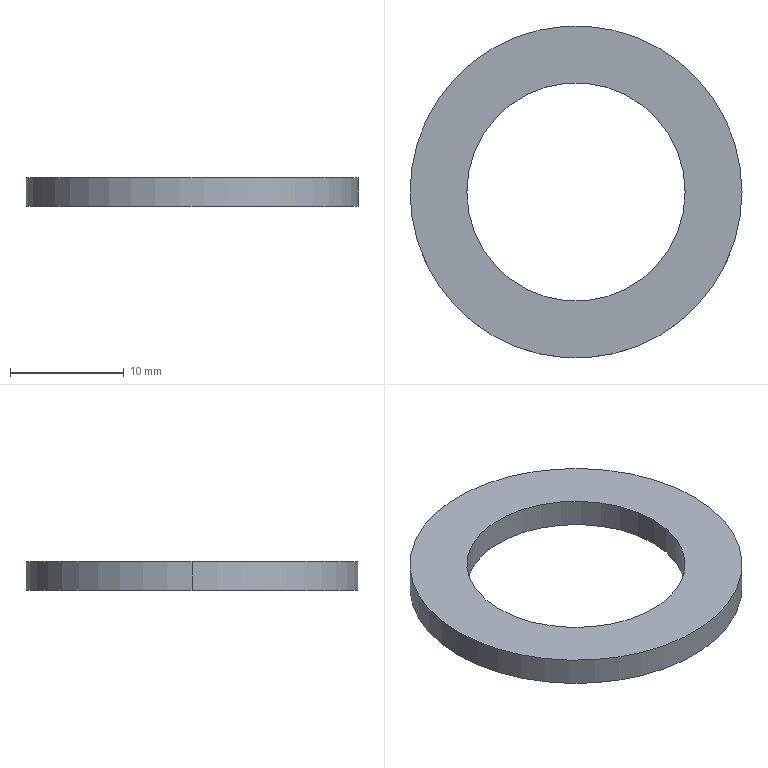Component | SolidWorks | TractionDrivenWheel-1_BearingPlate2-1 | 1 solid | 6 faces | box 29.2 x 29.2 x 2.5 mm | volume 950 mm3 | cylinder 4 | plane 2 | commonest cylinder face diameters 19.2 x2 29.2 x2
build123d program:
from build123d import *

# Parameters (mm, degrees)
SKETCH1_R           = 14.6
SKETCH1_R_2         = 9.6
BOSS_EXTRUDE1_DEPTH = 2.5


with BuildPart() as part:
    # Sketch1 → Boss-Extrude1 (new body)
    with BuildSketch(Plane(origin=(0, 0, 0), x_dir=(0, 0, -1), z_dir=(1, 0, 0))):
        Circle(SKETCH1_R)
        Circle(SKETCH1_R_2, mode=Mode.SUBTRACT)
    extrude(amount=BOSS_EXTRUDE1_DEPTH)


solid = part.part

# Placed as in the assembly
solid = solid.moved(Location((225.493, -197.911, 521), (0, 90, 0)))
STEP:
#1=CARTESIAN_POINT('',(9.256,-7.792,20.413));
#2=VERTEX_POINT('',#1);
#3=CARTESIAN_POINT('',(8.5,-7.792,20.413));
#4=VERTEX_POINT('',#3);
#5=CARTESIAN_POINT('',(8.878,-7.792,20.413));
#6=DIRECTION('',(0.,0.,-1.));
#7=DIRECTION('',(-1.,0.,0.));
#8=AXIS2_PLACEMENT_3D('',#5,#6,#7);
#9=CIRCLE('',#8,0.378);
#10=EDGE_CURVE('',#2,#4,#9,.T.);
#11=ORIENTED_EDGE('',*,*,#10,.T.);
#12=CARTESIAN_POINT('',(8.5,-7.792,20.512));
#13=VERTEX_POINT('',#12);
#14=CARTESIAN_POINT('',(8.5,-7.792,20.413));
#15=DIRECTION('',(0.,0.,1.));
#16=VECTOR('',#15,39.37);
#17=LINE('',#14,#16);
#18=EDGE_CURVE('',#4,#13,#17,.T.);
#19=ORIENTED_EDGE('',*,*,#18,.T.);
#20=CARTESIAN_POINT('',(9.256,-7.792,20.512));
#21=VERTEX_POINT('',#20);
#22=CARTESIAN_POINT('',(8.878,-7.792,20.512));
#23=DIRECTION('',(0.,0.,-1.));
#24=DIRECTION('',(-1.,0.,0.));
#25=AXIS2_PLACEMENT_3D('',#22,#23,#24);
#26=CIRCLE('',#25,0.378);
#27=EDGE_CURVE('',#21,#13,#26,.T.);
#28=ORIENTED_EDGE('',*,*,#27,.F.);
#29=CARTESIAN_POINT('',(9.256,-7.792,20.413));
#30=DIRECTION('',(0.,0.,1.));
#31=VECTOR('',#30,39.37);
#32=LINE('',#29,#31);
#33=EDGE_CURVE('',#2,#21,#32,.T.);
#34=ORIENTED_EDGE('',*,*,#33,.F.);
#35=EDGE_LOOP('',(#11,#19,#28,#34));
#36=FACE_OUTER_BOUND('',#35,.T.);
#37=CARTESIAN_POINT('',(8.878,-7.792,20.413));
#38=DIRECTION('',(0.,0.,1.));
#39=DIRECTION('',(1.,0.,0.));
#40=AXIS2_PLACEMENT_3D('',#37,#38,#39);
#41=CYLINDRICAL_SURFACE('',#40,0.378);
#42=ADVANCED_FACE('',(#36),#41,.F.);
#43=CARTESIAN_POINT('',(8.303,-7.792,20.413));
#44=VERTEX_POINT('',#43);
#45=CARTESIAN_POINT('',(9.452,-7.792,20.413));
#46=VERTEX_POINT('',#45);
#47=CARTESIAN_POINT('',(8.878,-7.792,20.413));
#48=DIRECTION('',(0.,0.,-1.));
#49=DIRECTION('',(-1.,0.,0.));
#50=AXIS2_PLACEMENT_3D('',#47,#48,#49);
#51=CIRCLE('',#50,0.5748);
#52=EDGE_CURVE('',#44,#46,#51,.T.);
#53=ORIENTED_EDGE('',*,*,#52,.F.);
#54=CARTESIAN_POINT('',(8.303,-7.792,20.512));
#55=VERTEX_POINT('',#54);
#56=CARTESIAN_POINT('',(8.303,-7.792,20.413));
#57=DIRECTION('',(0.,0.,1.));
#58=VECTOR('',#57,39.37);
#59=LINE('',#56,#58);
#60=EDGE_CURVE('',#44,#55,#59,.T.);
#61=ORIENTED_EDGE('',*,*,#60,.T.);
#62=CARTESIAN_POINT('',(9.452,-7.792,20.512));
#63=VERTEX_POINT('',#62);
#64=CARTESIAN_POINT('',(8.878,-7.792,20.512));
#65=DIRECTION('',(0.,0.,-1.));
#66=DIRECTION('',(-1.,0.,0.));
#67=AXIS2_PLACEMENT_3D('',#64,#65,#66);
#68=CIRCLE('',#67,0.5748);
#69=EDGE_CURVE('',#55,#63,#68,.T.);
#70=ORIENTED_EDGE('',*,*,#69,.T.);
#71=CARTESIAN_POINT('',(9.452,-7.792,20.413));
#72=DIRECTION('',(0.,0.,1.));
#73=VECTOR('',#72,39.37);
#74=LINE('',#71,#73);
#75=EDGE_CURVE('',#46,#63,#74,.T.);
#76=ORIENTED_EDGE('',*,*,#75,.F.);
#77=EDGE_LOOP('',(#53,#61,#70,#76));
#78=FACE_OUTER_BOUND('',#77,.T.);
#79=CARTESIAN_POINT('',(8.878,-7.792,20.413));
#80=DIRECTION('',(0.,0.,1.));
#81=DIRECTION('',(1.,0.,0.));
#82=AXIS2_PLACEMENT_3D('',#79,#80,#81);
#83=CYLINDRICAL_SURFACE('',#82,0.5748);
#84=ADVANCED_FACE('',(#78),#83,.T.);
#85=CARTESIAN_POINT('',(8.878,-7.792,20.413));
#86=DIRECTION('',(0.,0.,-1.));
#87=DIRECTION('',(-1.,0.,0.));
#88=AXIS2_PLACEMENT_3D('',#85,#86,#87);
#89=CIRCLE('',#88,0.5748);
#90=EDGE_CURVE('',#46,#44,#89,.T.);
#91=ORIENTED_EDGE('',*,*,#90,.T.);
#92=ORIENTED_EDGE('',*,*,#52,.T.);
#93=EDGE_LOOP('',(#91,#92));
#94=FACE_OUTER_BOUND('',#93,.T.);
#95=ORIENTED_EDGE('',*,*,#10,.F.);
#96=CARTESIAN_POINT('',(8.878,-7.792,20.413));
#97=DIRECTION('',(0.,0.,-1.));
#98=DIRECTION('',(-1.,0.,0.));
#99=AXIS2_PLACEMENT_3D('',#96,#97,#98);
#100=CIRCLE('',#99,0.378);
#101=EDGE_CURVE('',#4,#2,#100,.T.);
#102=ORIENTED_EDGE('',*,*,#101,.F.);
#103=EDGE_LOOP('',(#95,#102));
#104=FACE_BOUND('',#103,.T.);
#105=CARTESIAN_POINT('',(8.878,-7.792,20.413));
#106=DIRECTION('',(0.,0.,-1.));
#107=DIRECTION('',(-1.,-0.,0.));
#108=AXIS2_PLACEMENT_3D('',#105,#106,#107);
#109=PLANE('',#108);
#110=ADVANCED_FACE('',(#94,#104),#109,.T.);
#111=CARTESIAN_POINT('',(8.878,-7.792,20.512));
#112=DIRECTION('',(0.,0.,-1.));
#113=DIRECTION('',(-1.,0.,0.));
#114=AXIS2_PLACEMENT_3D('',#111,#112,#113);
#115=CIRCLE('',#114,0.5748);
#116=EDGE_CURVE('',#63,#55,#115,.T.);
#117=ORIENTED_EDGE('',*,*,#116,.F.);
#118=ORIENTED_EDGE('',*,*,#69,.F.);
#119=EDGE_LOOP('',(#117,#118));
#120=FACE_OUTER_BOUND('',#119,.T.);
#121=ORIENTED_EDGE('',*,*,#27,.T.);
#122=CARTESIAN_POINT('',(8.878,-7.792,20.512));
#123=DIRECTION('',(0.,0.,-1.));
#124=DIRECTION('',(-1.,0.,0.));
#125=AXIS2_PLACEMENT_3D('',#122,#123,#124);
#126=CIRCLE('',#125,0.378);
#127=EDGE_CURVE('',#13,#21,#126,.T.);
#128=ORIENTED_EDGE('',*,*,#127,.T.);
#129=EDGE_LOOP('',(#121,#128));
#130=FACE_BOUND('',#129,.T.);
#131=CARTESIAN_POINT('',(8.878,-7.792,20.512));
#132=DIRECTION('',(0.,0.,-1.));
#133=DIRECTION('',(-1.,-0.,0.));
#134=AXIS2_PLACEMENT_3D('',#131,#132,#133);
#135=PLANE('',#134);
#136=ADVANCED_FACE('',(#120,#130),#135,.F.);
#137=ORIENTED_EDGE('',*,*,#60,.F.);
#138=ORIENTED_EDGE('',*,*,#90,.F.);
#139=ORIENTED_EDGE('',*,*,#75,.T.);
#140=ORIENTED_EDGE('',*,*,#116,.T.);
#141=EDGE_LOOP('',(#137,#138,#139,#140));
#142=FACE_OUTER_BOUND('',#141,.T.);
#143=CARTESIAN_POINT('',(8.878,-7.792,20.413));
#144=DIRECTION('',(0.,0.,1.));
#145=DIRECTION('',(1.,0.,0.));
#146=AXIS2_PLACEMENT_3D('',#143,#144,#145);
#147=CYLINDRICAL_SURFACE('',#146,0.5748);
#148=ADVANCED_FACE('',(#142),#147,.T.);
#149=ORIENTED_EDGE('',*,*,#18,.F.);
#150=ORIENTED_EDGE('',*,*,#101,.T.);
#151=ORIENTED_EDGE('',*,*,#33,.T.);
#152=ORIENTED_EDGE('',*,*,#127,.F.);
#153=EDGE_LOOP('',(#149,#150,#151,#152));
#154=FACE_OUTER_BOUND('',#153,.T.);
#155=CARTESIAN_POINT('',(8.878,-7.792,20.413));
#156=DIRECTION('',(0.,0.,1.));
#157=DIRECTION('',(1.,0.,0.));
#158=AXIS2_PLACEMENT_3D('',#155,#156,#157);
#159=CYLINDRICAL_SURFACE('',#158,0.378);
#160=ADVANCED_FACE('',(#154),#159,.F.);
#161=CLOSED_SHELL('',(#42,#84,#110,#136,#148,#160));
#162=MANIFOLD_SOLID_BREP('',#161);
#163=CARTESIAN_POINT('',(0.,0.,0.));
#164=DIRECTION('',(0.,0.,1.));
#165=DIRECTION('',(1.,0.,0.));
#166=AXIS2_PLACEMENT_3D('',#163,#164,#165);
#167=(LENGTH_UNIT()NAMED_UNIT(*)SI_UNIT($,.METRE.));
#168=LENGTH_MEASURE_WITH_UNIT(LENGTH_MEASURE(0.0254),#167);
#169=DIMENSIONAL_EXPONENTS(1.,0.,0.,0.,0.,0.,0.);
#170=(CONVERSION_BASED_UNIT('',#168)LENGTH_UNIT()NAMED_UNIT(#169));
#171=UNCERTAINTY_MEASURE_WITH_UNIT(LENGTH_MEASURE(0.00001),#170,'','');
#172=(NAMED_UNIT(*)PLANE_ANGLE_UNIT()SI_UNIT($,.RADIAN.));
#173=(NAMED_UNIT(*)SI_UNIT($,.STERADIAN.)SOLID_ANGLE_UNIT());
#174=(GEOMETRIC_REPRESENTATION_CONTEXT(3)GLOBAL_UNCERTAINTY_ASSIGNED_CONTEXT((#171))GLOBAL_UNIT_ASSIGNED_CONTEXT((#170,#172,#173))REPRESENTATION_CONTEXT('',''));
#175=ADVANCED_BREP_SHAPE_REPRESENTATION('',(#162,#166),#174);
#176=COLOUR_RGB('',0.7922,0.8196,0.9333);
#177=FILL_AREA_STYLE_COLOUR('',#176);
#178=FILL_AREA_STYLE('',(#177));
#179=SURFACE_STYLE_FILL_AREA(#178);
#180=SURFACE_SIDE_STYLE('',(#179));
#181=SURFACE_STYLE_USAGE(.BOTH.,#180);
#182=PRESENTATION_STYLE_ASSIGNMENT((#181));
#183=STYLED_ITEM('',(#182),#162);
#184=(LENGTH_UNIT()NAMED_UNIT(*)SI_UNIT($,.METRE.));
#185=LENGTH_MEASURE_WITH_UNIT(LENGTH_MEASURE(0.0254),#184);
#186=DIMENSIONAL_EXPONENTS(1.,0.,0.,0.,0.,0.,0.);
#187=(CONVERSION_BASED_UNIT('',#185)LENGTH_UNIT()NAMED_UNIT(#186));
#188=UNCERTAINTY_MEASURE_WITH_UNIT(LENGTH_MEASURE(0.00001),#187,'','');
#189=(NAMED_UNIT(*)PLANE_ANGLE_UNIT()SI_UNIT($,.RADIAN.));
#190=(NAMED_UNIT(*)SI_UNIT($,.STERADIAN.)SOLID_ANGLE_UNIT());
#191=(GEOMETRIC_REPRESENTATION_CONTEXT(3)GLOBAL_UNCERTAINTY_ASSIGNED_CONTEXT((#188))GLOBAL_UNIT_ASSIGNED_CONTEXT((#187,#189,#190))REPRESENTATION_CONTEXT('',''));
#192=MECHANICAL_DESIGN_GEOMETRIC_PRESENTATION_REPRESENTATION('',(#183),#191);
#193=PRESENTATION_LAYER_ASSIGNMENT('','',(#183));